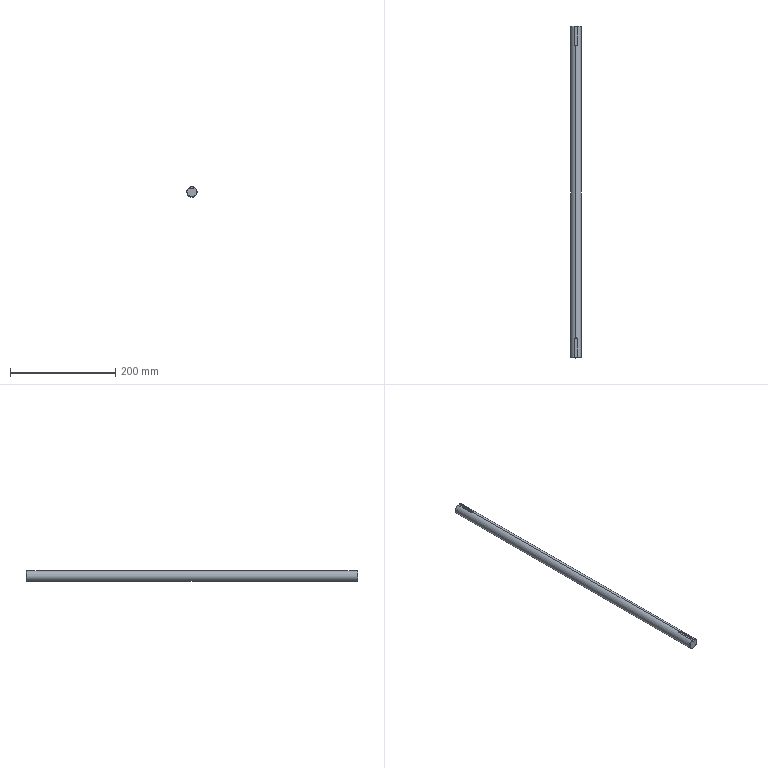Component | SolidWorks | ZL-11-09DriveShaft2-1 | 1 solid | 15 faces | box 20 x 630 x 20 mm | volume 196364 mm3 | plane 8 | cylinder 4 | cone 3 | commonest cylinder face diameters 20 x2 6 x2
build123d program:
from build123d import *

# Parameters (mm, degrees)
SKETCH1_R          = 10
EXTRUDE1_DEPTH     = 315
CUT_EXTRUDE1_DEPTH = 3.5
CHAMFER1_SIZE      = 1


with BuildPart() as part:
    # Sketch1 → Extrude1 (new, symmetric)
    with BuildSketch(Plane(origin=(0, 0, 0), x_dir=(1, 0, 0), z_dir=(0, 1, 0))):
        with Locations(Location((0, 0, 0), (0, 0, 270))):
            Circle(SKETCH1_R)
    extrude(amount=EXTRUDE1_DEPTH, both=True)

    # Sketch2 → Cut-Extrude1 (cut)
    with BuildSketch(Plane.XY.offset(10)):
        with BuildLine():
            Line((-3, 315), (3, 315))
            Line((3, 315), (3, 280))
            ThreePointArc((3, 280), (0, 277), (-3, 280))
            Line((-3, 280), (-3, 315))
        make_face()
    cut_extrude1 = extrude(amount=-CUT_EXTRUDE1_DEPTH, mode=Mode.SUBTRACT)

    # Mirror1: Cut-Extrude1 across plane
    add(cut_extrude1.mirror(Plane.ZX), mode=Mode.SUBTRACT)

    # Chamfer1
    chamfer1_edges = [part.edges().sort_by_distance(p)[0] for p in [
        (0, -315, -10),
        (0, 315, -10),
    ]]
    chamfer(chamfer1_edges, length=CHAMFER1_SIZE)


solid = part.part

# Placed as in the assembly
solid = solid.moved(Location((125.552, 443.22, 0.7679), (0, -1.419, 180)))
STEP:
#1=COLOUR_RGB('',0.7922,0.8196,0.9333);
#2=FILL_AREA_STYLE_COLOUR('',#1);
#3=FILL_AREA_STYLE('',(#2));
#4=SURFACE_STYLE_FILL_AREA(#3);
#5=SURFACE_SIDE_STYLE('',(#4));
#6=SURFACE_STYLE_USAGE(.BOTH.,#5);
#7=PRESENTATION_STYLE_ASSIGNMENT((#6));
#8=CARTESIAN_POINT('',(4.952,29.851,-0.324));
#9=VERTEX_POINT('',#8);
#10=CARTESIAN_POINT('',(4.817,29.851,0.3613));
#11=VERTEX_POINT('',#10);
#12=CARTESIAN_POINT('',(4.943,29.851,0.03023));
#13=DIRECTION('',(0.,1.,0.));
#14=DIRECTION('',(-0.02476,0.,0.9997));
#15=AXIS2_PLACEMENT_3D('',#12,#13,#14);
#16=CIRCLE('',#15,0.3543);
#17=EDGE_CURVE('',#9,#11,#16,.T.);
#18=ORIENTED_EDGE('',*,*,#17,.F.);
#19=CARTESIAN_POINT('',(4.953,29.812,-0.3633));
#20=VERTEX_POINT('',#19);
#21=CARTESIAN_POINT('',(4.952,29.851,-0.324));
#22=DIRECTION('',(0.01751,-0.7071,-0.7069));
#23=VECTOR('',#22,39.37);
#24=LINE('',#21,#23);
#25=EDGE_CURVE('',#9,#20,#24,.T.);
#26=ORIENTED_EDGE('',*,*,#25,.T.);
#27=CARTESIAN_POINT('',(4.816,29.812,0.4028));
#28=VERTEX_POINT('',#27);
#29=CARTESIAN_POINT('',(4.943,29.812,0.03023));
#30=DIRECTION('',(0.,-1.,0.));
#31=DIRECTION('',(-0.02476,0.,0.9997));
#32=AXIS2_PLACEMENT_3D('',#29,#30,#31);
#33=CIRCLE('',#32,0.3937);
#34=EDGE_CURVE('',#28,#20,#33,.T.);
#35=ORIENTED_EDGE('',*,*,#34,.F.);
#36=CARTESIAN_POINT('',(4.817,29.851,0.3613));
#37=CARTESIAN_POINT('',(4.816,29.838,0.3751));
#38=CARTESIAN_POINT('',(4.816,29.825,0.389));
#39=CARTESIAN_POINT('',(4.816,29.812,0.4028));
#40=B_SPLINE_CURVE_WITH_KNOTS('',3,(#36,#37,#38,#39),.UNSPECIFIED.,.F.,.F.,(4,4),(0.,0.001453),.UNSPECIFIED.);
#41=EDGE_CURVE('',#11,#28,#40,.T.);
#42=ORIENTED_EDGE('',*,*,#41,.F.);
#43=EDGE_LOOP('',(#18,#26,#35,#42));
#44=FACE_OUTER_BOUND('',#43,.T.);
#45=CARTESIAN_POINT('',(4.943,29.851,0.03023));
#46=DIRECTION('',(0.,-1.,0.));
#47=DIRECTION('',(0.02476,0.,-0.9997));
#48=AXIS2_PLACEMENT_3D('',#45,#46,#47);
#49=CONICAL_SURFACE('',#48,0.3543,0.7854);
#50=ADVANCED_FACE('',(#44),#49,.T.);
#51=CARTESIAN_POINT('',(5.052,28.473,0.4086));
#52=VERTEX_POINT('',#51);
#53=CARTESIAN_POINT('',(4.933,28.355,0.4238));
#54=VERTEX_POINT('',#53);
#55=CARTESIAN_POINT('',(5.052,28.473,0.4086));
#56=CARTESIAN_POINT('',(5.052,28.465,0.4086));
#57=CARTESIAN_POINT('',(5.051,28.458,0.4088));
#58=CARTESIAN_POINT('',(5.048,28.442,0.4097));
#59=CARTESIAN_POINT('',(5.046,28.435,0.4103));
#60=CARTESIAN_POINT('',(5.04,28.421,0.4119));
#61=CARTESIAN_POINT('',(5.036,28.414,0.4128));
#62=CARTESIAN_POINT('',(5.027,28.401,0.4148));
#63=CARTESIAN_POINT('',(5.022,28.395,0.4159));
#64=CARTESIAN_POINT('',(5.006,28.379,0.419));
#65=CARTESIAN_POINT('',(4.993,28.37,0.421));
#66=CARTESIAN_POINT('',(4.972,28.361,0.423));
#67=CARTESIAN_POINT('',(4.964,28.359,0.4234));
#68=CARTESIAN_POINT('',(4.949,28.356,0.424));
#69=CARTESIAN_POINT('',(4.941,28.355,0.424));
#70=CARTESIAN_POINT('',(4.933,28.355,0.4238));
#71=B_SPLINE_CURVE_WITH_KNOTS('',3,(#55,#56,#57,#58,#59,#60,#61,#62,#63,#64,#65,#66,#67,#68,#69,#70),.UNSPECIFIED.,.F.,.F.,(4,2,2,2,2,2,2,4),(0.,0.0005898,0.00118,0.001769,0.002359,0.003539,0.004128,0.004718),.UNSPECIFIED.);
#72=EDGE_CURVE('',#52,#54,#71,.T.);
#73=ORIENTED_EDGE('',*,*,#72,.T.);
#74=CARTESIAN_POINT('',(4.933,6.544,0.4238));
#75=VERTEX_POINT('',#74);
#76=CARTESIAN_POINT('',(4.933,29.851,0.4238));
#77=DIRECTION('',(0.,-1.,0.));
#78=VECTOR('',#77,39.37);
#79=LINE('',#76,#78);
#80=EDGE_CURVE('',#54,#75,#79,.T.);
#81=ORIENTED_EDGE('',*,*,#80,.T.);
#82=CARTESIAN_POINT('',(5.052,6.426,0.4086));
#83=VERTEX_POINT('',#82);
#84=CARTESIAN_POINT('',(5.052,6.426,0.4086));
#85=CARTESIAN_POINT('',(5.052,6.434,0.4086));
#86=CARTESIAN_POINT('',(5.051,6.442,0.4088));
#87=CARTESIAN_POINT('',(5.048,6.457,0.4097));
#88=CARTESIAN_POINT('',(5.046,6.464,0.4103));
#89=CARTESIAN_POINT('',(5.04,6.479,0.4119));
#90=CARTESIAN_POINT('',(5.036,6.485,0.4128));
#91=CARTESIAN_POINT('',(5.027,6.498,0.4148));
#92=CARTESIAN_POINT('',(5.022,6.504,0.4159));
#93=CARTESIAN_POINT('',(5.006,6.52,0.419));
#94=CARTESIAN_POINT('',(4.993,6.529,0.421));
#95=CARTESIAN_POINT('',(4.972,6.538,0.423));
#96=CARTESIAN_POINT('',(4.964,6.54,0.4234));
#97=CARTESIAN_POINT('',(4.949,6.543,0.424));
#98=CARTESIAN_POINT('',(4.941,6.544,0.424));
#99=CARTESIAN_POINT('',(4.933,6.544,0.4238));
#100=B_SPLINE_CURVE_WITH_KNOTS('',3,(#84,#85,#86,#87,#88,#89,#90,#91,#92,#93,#94,#95,#96,#97,#98,#99),.UNSPECIFIED.,.F.,.F.,(4,2,2,2,2,2,2,4),(0.,0.0005898,0.00118,0.001769,0.002359,0.003539,0.004128,0.004718),.UNSPECIFIED.);
#101=EDGE_CURVE('',#83,#75,#100,.T.);
#102=ORIENTED_EDGE('',*,*,#101,.F.);
#103=CARTESIAN_POINT('',(5.052,5.087,0.4086));
#104=VERTEX_POINT('',#103);
#105=CARTESIAN_POINT('',(5.052,29.851,0.4086));
#106=DIRECTION('',(0.,1.,0.));
#107=VECTOR('',#106,39.37);
#108=LINE('',#105,#107);
#109=EDGE_CURVE('',#104,#83,#108,.T.);
#110=ORIENTED_EDGE('',*,*,#109,.F.);
#111=CARTESIAN_POINT('',(4.953,5.087,-0.3633));
#112=VERTEX_POINT('',#111);
#113=CARTESIAN_POINT('',(4.943,5.087,0.03023));
#114=DIRECTION('',(0.,1.,0.));
#115=DIRECTION('',(-0.02476,0.,0.9997));
#116=AXIS2_PLACEMENT_3D('',#113,#114,#115);
#117=CIRCLE('',#116,0.3937);
#118=EDGE_CURVE('',#104,#112,#117,.T.);
#119=ORIENTED_EDGE('',*,*,#118,.T.);
#120=CARTESIAN_POINT('',(4.953,29.851,-0.3633));
#121=DIRECTION('',(0.,-1.,0.));
#122=VECTOR('',#121,39.37);
#123=LINE('',#120,#122);
#124=EDGE_CURVE('',#20,#112,#123,.T.);
#125=ORIENTED_EDGE('',*,*,#124,.F.);
#126=CARTESIAN_POINT('',(5.052,29.812,0.4086));
#127=VERTEX_POINT('',#126);
#128=CARTESIAN_POINT('',(4.943,29.812,0.03023));
#129=DIRECTION('',(0.,-1.,0.));
#130=DIRECTION('',(-0.02476,0.,0.9997));
#131=AXIS2_PLACEMENT_3D('',#128,#129,#130);
#132=CIRCLE('',#131,0.3937);
#133=EDGE_CURVE('',#20,#127,#132,.T.);
#134=ORIENTED_EDGE('',*,*,#133,.T.);
#135=CARTESIAN_POINT('',(5.052,29.851,0.4086));
#136=DIRECTION('',(0.,-1.,0.));
#137=VECTOR('',#136,39.37);
#138=LINE('',#135,#137);
#139=EDGE_CURVE('',#127,#52,#138,.T.);
#140=ORIENTED_EDGE('',*,*,#139,.T.);
#141=EDGE_LOOP('',(#73,#81,#102,#110,#119,#125,#134,#140));
#142=FACE_OUTER_BOUND('',#141,.T.);
#143=CARTESIAN_POINT('',(4.943,29.851,0.03023));
#144=DIRECTION('',(0.,-1.,0.));
#145=DIRECTION('',(0.02476,0.,-0.9997));
#146=AXIS2_PLACEMENT_3D('',#143,#144,#145);
#147=CYLINDRICAL_SURFACE('',#146,0.3937);
#148=ADVANCED_FACE('',(#142),#147,.T.);
#149=ORIENTED_EDGE('',*,*,#80,.F.);
#150=CARTESIAN_POINT('',(4.816,28.473,0.4028));
#151=VERTEX_POINT('',#150);
#152=CARTESIAN_POINT('',(4.933,28.355,0.4238));
#153=CARTESIAN_POINT('',(4.925,28.355,0.4236));
#154=CARTESIAN_POINT('',(4.918,28.356,0.4232));
#155=CARTESIAN_POINT('',(4.902,28.359,0.4219));
#156=CARTESIAN_POINT('',(4.895,28.361,0.4211));
#157=CARTESIAN_POINT('',(4.881,28.367,0.4191));
#158=CARTESIAN_POINT('',(4.874,28.371,0.4179));
#159=CARTESIAN_POINT('',(4.861,28.379,0.4154));
#160=CARTESIAN_POINT('',(4.855,28.384,0.4141));
#161=CARTESIAN_POINT('',(4.845,28.395,0.4115));
#162=CARTESIAN_POINT('',(4.84,28.401,0.4102));
#163=CARTESIAN_POINT('',(4.831,28.414,0.4078));
#164=CARTESIAN_POINT('',(4.828,28.421,0.4066));
#165=CARTESIAN_POINT('',(4.822,28.435,0.4048));
#166=CARTESIAN_POINT('',(4.819,28.442,0.404));
#167=CARTESIAN_POINT('',(4.816,28.458,0.403));
#168=CARTESIAN_POINT('',(4.816,28.465,0.4028));
#169=CARTESIAN_POINT('',(4.816,28.473,0.4028));
#170=B_SPLINE_CURVE_WITH_KNOTS('',3,(#152,#153,#154,#155,#156,#157,#158,#159,#160,#161,#162,#163,#164,#165,#166,#167,#168,#169),.UNSPECIFIED.,.F.,.F.,(4,2,2,2,2,2,2,2,4),(0.004718,0.005307,0.005896,0.006485,0.007074,0.007663,0.008252,0.008842,0.009431),.UNSPECIFIED.);
#171=EDGE_CURVE('',#54,#151,#170,.T.);
#172=ORIENTED_EDGE('',*,*,#171,.T.);
#173=CARTESIAN_POINT('',(4.816,29.851,0.4028));
#174=DIRECTION('',(0.,1.,0.));
#175=VECTOR('',#174,39.37);
#176=LINE('',#173,#175);
#177=EDGE_CURVE('',#151,#28,#176,.T.);
#178=ORIENTED_EDGE('',*,*,#177,.T.);
#179=ORIENTED_EDGE('',*,*,#34,.T.);
#180=ORIENTED_EDGE('',*,*,#124,.T.);
#181=CARTESIAN_POINT('',(4.816,5.087,0.4028));
#182=VERTEX_POINT('',#181);
#183=CARTESIAN_POINT('',(4.943,5.087,0.03023));
#184=DIRECTION('',(0.,1.,0.));
#185=DIRECTION('',(-0.02476,0.,0.9997));
#186=AXIS2_PLACEMENT_3D('',#183,#184,#185);
#187=CIRCLE('',#186,0.3937);
#188=EDGE_CURVE('',#112,#182,#187,.T.);
#189=ORIENTED_EDGE('',*,*,#188,.T.);
#190=CARTESIAN_POINT('',(4.816,6.426,0.4028));
#191=VERTEX_POINT('',#190);
#192=CARTESIAN_POINT('',(4.816,29.851,0.4028));
#193=DIRECTION('',(0.,-1.,0.));
#194=VECTOR('',#193,39.37);
#195=LINE('',#192,#194);
#196=EDGE_CURVE('',#191,#182,#195,.T.);
#197=ORIENTED_EDGE('',*,*,#196,.F.);
#198=CARTESIAN_POINT('',(4.933,6.544,0.4238));
#199=CARTESIAN_POINT('',(4.925,6.544,0.4236));
#200=CARTESIAN_POINT('',(4.918,6.543,0.4232));
#201=CARTESIAN_POINT('',(4.902,6.54,0.4219));
#202=CARTESIAN_POINT('',(4.895,6.538,0.4211));
#203=CARTESIAN_POINT('',(4.881,6.532,0.4191));
#204=CARTESIAN_POINT('',(4.874,6.528,0.4179));
#205=CARTESIAN_POINT('',(4.861,6.52,0.4154));
#206=CARTESIAN_POINT('',(4.855,6.515,0.4141));
#207=CARTESIAN_POINT('',(4.845,6.504,0.4115));
#208=CARTESIAN_POINT('',(4.84,6.498,0.4102));
#209=CARTESIAN_POINT('',(4.831,6.485,0.4078));
#210=CARTESIAN_POINT('',(4.828,6.478,0.4066));
#211=CARTESIAN_POINT('',(4.822,6.464,0.4048));
#212=CARTESIAN_POINT('',(4.819,6.457,0.404));
#213=CARTESIAN_POINT('',(4.816,6.442,0.403));
#214=CARTESIAN_POINT('',(4.816,6.434,0.4028));
#215=CARTESIAN_POINT('',(4.816,6.426,0.4028));
#216=B_SPLINE_CURVE_WITH_KNOTS('',3,(#198,#199,#200,#201,#202,#203,#204,#205,#206,#207,#208,#209,#210,#211,#212,#213,#214,#215),.UNSPECIFIED.,.F.,.F.,(4,2,2,2,2,2,2,2,4),(0.004718,0.005307,0.005896,0.006485,0.007074,0.007663,0.008252,0.008842,0.009431),.UNSPECIFIED.);
#217=EDGE_CURVE('',#75,#191,#216,.T.);
#218=ORIENTED_EDGE('',*,*,#217,.F.);
#219=EDGE_LOOP('',(#149,#172,#178,#179,#180,#189,#197,#218));
#220=FACE_OUTER_BOUND('',#219,.T.);
#221=CARTESIAN_POINT('',(4.943,29.851,0.03023));
#222=DIRECTION('',(0.,-1.,0.));
#223=DIRECTION('',(0.02476,0.,-0.9997));
#224=AXIS2_PLACEMENT_3D('',#221,#222,#223);
#225=CYLINDRICAL_SURFACE('',#224,0.3937);
#226=ADVANCED_FACE('',(#220),#225,.T.);
#227=CARTESIAN_POINT('',(4.819,5.048,0.2831));
#228=VERTEX_POINT('',#227);
#229=CARTESIAN_POINT('',(4.817,5.048,0.3613));
#230=VERTEX_POINT('',#229);
#231=CARTESIAN_POINT('',(4.819,5.048,0.2831));
#232=DIRECTION('',(-0.02476,0.,0.9997));
#233=VECTOR('',#232,39.37);
#234=LINE('',#231,#233);
#235=EDGE_CURVE('',#228,#230,#234,.T.);
#236=ORIENTED_EDGE('',*,*,#235,.T.);
#237=CARTESIAN_POINT('',(5.053,5.048,0.3671));
#238=VERTEX_POINT('',#237);
#239=CARTESIAN_POINT('',(4.943,5.048,0.03023));
#240=DIRECTION('',(0.,-1.,0.));
#241=DIRECTION('',(-0.02476,0.,0.9997));
#242=AXIS2_PLACEMENT_3D('',#239,#240,#241);
#243=CIRCLE('',#242,0.3543);
#244=EDGE_CURVE('',#230,#238,#243,.T.);
#245=ORIENTED_EDGE('',*,*,#244,.T.);
#246=CARTESIAN_POINT('',(5.055,5.048,0.289));
#247=VERTEX_POINT('',#246);
#248=CARTESIAN_POINT('',(5.055,5.048,0.289));
#249=DIRECTION('',(-0.02476,0.,0.9997));
#250=VECTOR('',#249,39.37);
#251=LINE('',#248,#250);
#252=EDGE_CURVE('',#247,#238,#251,.T.);
#253=ORIENTED_EDGE('',*,*,#252,.F.);
#254=CARTESIAN_POINT('',(4.819,5.048,0.2831));
#255=DIRECTION('',(-0.9997,0.,-0.02476));
#256=VECTOR('',#255,39.37);
#257=LINE('',#254,#256);
#258=EDGE_CURVE('',#247,#228,#257,.T.);
#259=ORIENTED_EDGE('',*,*,#258,.T.);
#260=EDGE_LOOP('',(#236,#245,#253,#259));
#261=FACE_OUTER_BOUND('',#260,.T.);
#262=CARTESIAN_POINT('',(4.943,5.048,0.03023));
#263=DIRECTION('',(0.,1.,0.));
#264=DIRECTION('',(-0.02476,0.,0.9997));
#265=AXIS2_PLACEMENT_3D('',#262,#263,#264);
#266=PLANE('',#265);
#267=ADVANCED_FACE('',(#261),#266,.F.);
#268=CARTESIAN_POINT('',(5.055,29.851,0.289));
#269=VERTEX_POINT('',#268);
#270=CARTESIAN_POINT('',(5.053,29.851,0.3671));
#271=VERTEX_POINT('',#270);
#272=CARTESIAN_POINT('',(5.055,29.851,0.289));
#273=DIRECTION('',(-0.02476,0.,0.9997));
#274=VECTOR('',#273,39.37);
#275=LINE('',#272,#274);
#276=EDGE_CURVE('',#269,#271,#275,.T.);
#277=ORIENTED_EDGE('',*,*,#276,.T.);
#278=CARTESIAN_POINT('',(4.943,29.851,0.03023));
#279=DIRECTION('',(0.,1.,0.));
#280=DIRECTION('',(-0.02476,0.,0.9997));
#281=AXIS2_PLACEMENT_3D('',#278,#279,#280);
#282=CIRCLE('',#281,0.3543);
#283=EDGE_CURVE('',#271,#9,#282,.T.);
#284=ORIENTED_EDGE('',*,*,#283,.T.);
#285=ORIENTED_EDGE('',*,*,#17,.T.);
#286=CARTESIAN_POINT('',(4.819,29.851,0.2831));
#287=VERTEX_POINT('',#286);
#288=CARTESIAN_POINT('',(4.819,29.851,0.2831));
#289=DIRECTION('',(-0.02476,0.,0.9997));
#290=VECTOR('',#289,39.37);
#291=LINE('',#288,#290);
#292=EDGE_CURVE('',#287,#11,#291,.T.);
#293=ORIENTED_EDGE('',*,*,#292,.F.);
#294=CARTESIAN_POINT('',(4.819,29.851,0.2831));
#295=DIRECTION('',(-0.9997,0.,-0.02476));
#296=VECTOR('',#295,39.37);
#297=LINE('',#294,#296);
#298=EDGE_CURVE('',#269,#287,#297,.T.);
#299=ORIENTED_EDGE('',*,*,#298,.F.);
#300=EDGE_LOOP('',(#277,#284,#285,#293,#299));
#301=FACE_OUTER_BOUND('',#300,.T.);
#302=CARTESIAN_POINT('',(4.943,29.851,0.03023));
#303=DIRECTION('',(0.,1.,0.));
#304=DIRECTION('',(-0.02476,0.,0.9997));
#305=AXIS2_PLACEMENT_3D('',#302,#303,#304);
#306=PLANE('',#305);
#307=ADVANCED_FACE('',(#301),#306,.T.);
#308=CARTESIAN_POINT('',(5.055,28.473,0.289));
#309=VERTEX_POINT('',#308);
#310=CARTESIAN_POINT('',(5.055,28.473,0.289));
#311=DIRECTION('',(-0.02476,0.,0.9997));
#312=VECTOR('',#311,39.37);
#313=LINE('',#310,#312);
#314=EDGE_CURVE('',#309,#52,#313,.T.);
#315=ORIENTED_EDGE('',*,*,#314,.F.);
#316=CARTESIAN_POINT('',(4.819,28.473,0.2831));
#317=VERTEX_POINT('',#316);
#318=CARTESIAN_POINT('',(4.937,28.473,0.2861));
#319=DIRECTION('',(-0.02476,0.,0.9997));
#320=DIRECTION('',(0.9997,0.,0.02476));
#321=AXIS2_PLACEMENT_3D('',#318,#319,#320);
#322=CIRCLE('',#321,0.1181);
#323=EDGE_CURVE('',#317,#309,#322,.T.);
#324=ORIENTED_EDGE('',*,*,#323,.F.);
#325=CARTESIAN_POINT('',(4.819,28.473,0.2831));
#326=DIRECTION('',(-0.02476,0.,0.9997));
#327=VECTOR('',#326,39.37);
#328=LINE('',#325,#327);
#329=EDGE_CURVE('',#317,#151,#328,.T.);
#330=ORIENTED_EDGE('',*,*,#329,.T.);
#331=ORIENTED_EDGE('',*,*,#171,.F.);
#332=ORIENTED_EDGE('',*,*,#72,.F.);
#333=EDGE_LOOP('',(#315,#324,#330,#331,#332));
#334=FACE_OUTER_BOUND('',#333,.T.);
#335=CARTESIAN_POINT('',(4.937,28.473,0.2861));
#336=DIRECTION('',(-0.02476,0.,0.9997));
#337=DIRECTION('',(0.9997,0.,0.02476));
#338=AXIS2_PLACEMENT_3D('',#335,#336,#337);
#339=CYLINDRICAL_SURFACE('',#338,0.1181);
#340=ADVANCED_FACE('',(#334),#339,.F.);
#341=ORIENTED_EDGE('',*,*,#292,.T.);
#342=ORIENTED_EDGE('',*,*,#41,.T.);
#343=ORIENTED_EDGE('',*,*,#177,.F.);
#344=ORIENTED_EDGE('',*,*,#329,.F.);
#345=CARTESIAN_POINT('',(4.819,29.851,0.2831));
#346=DIRECTION('',(0.,-1.,0.));
#347=VECTOR('',#346,39.37);
#348=LINE('',#345,#347);
#349=EDGE_CURVE('',#287,#317,#348,.T.);
#350=ORIENTED_EDGE('',*,*,#349,.F.);
#351=EDGE_LOOP('',(#341,#342,#343,#344,#350));
#352=FACE_OUTER_BOUND('',#351,.T.);
#353=CARTESIAN_POINT('',(4.819,29.851,0.2831));
#354=DIRECTION('',(-0.9997,-0.,-0.02476));
#355=DIRECTION('',(0.,-1.,0.));
#356=AXIS2_PLACEMENT_3D('',#353,#354,#355);
#357=PLANE('',#356);
#358=ADVANCED_FACE('',(#352),#357,.F.);
#359=ORIENTED_EDGE('',*,*,#139,.F.);
#360=CARTESIAN_POINT('',(5.052,29.812,0.4086));
#361=CARTESIAN_POINT('',(5.052,29.825,0.3948));
#362=CARTESIAN_POINT('',(5.052,29.838,0.381));
#363=CARTESIAN_POINT('',(5.053,29.851,0.3671));
#364=B_SPLINE_CURVE_WITH_KNOTS('',3,(#360,#361,#362,#363),.UNSPECIFIED.,.F.,.F.,(4,4),(0.,0.001453),.UNSPECIFIED.);
#365=EDGE_CURVE('',#127,#271,#364,.T.);
#366=ORIENTED_EDGE('',*,*,#365,.T.);
#367=ORIENTED_EDGE('',*,*,#276,.F.);
#368=CARTESIAN_POINT('',(5.055,29.851,0.289));
#369=DIRECTION('',(0.,1.,0.));
#370=VECTOR('',#369,39.37);
#371=LINE('',#368,#370);
#372=EDGE_CURVE('',#309,#269,#371,.T.);
#373=ORIENTED_EDGE('',*,*,#372,.F.);
#374=ORIENTED_EDGE('',*,*,#314,.T.);
#375=EDGE_LOOP('',(#359,#366,#367,#373,#374));
#376=FACE_OUTER_BOUND('',#375,.T.);
#377=CARTESIAN_POINT('',(5.055,29.851,0.289));
#378=DIRECTION('',(0.9997,-0.,0.02476));
#379=DIRECTION('',(0.,1.,0.));
#380=AXIS2_PLACEMENT_3D('',#377,#378,#379);
#381=PLANE('',#380);
#382=ADVANCED_FACE('',(#376),#381,.F.);
#383=ORIENTED_EDGE('',*,*,#349,.T.);
#384=ORIENTED_EDGE('',*,*,#323,.T.);
#385=ORIENTED_EDGE('',*,*,#372,.T.);
#386=ORIENTED_EDGE('',*,*,#298,.T.);
#387=EDGE_LOOP('',(#383,#384,#385,#386));
#388=FACE_OUTER_BOUND('',#387,.T.);
#389=CARTESIAN_POINT('',(4.937,28.473,0.2861));
#390=DIRECTION('',(-0.02476,0.,0.9997));
#391=DIRECTION('',(0.9997,0.,0.02476));
#392=AXIS2_PLACEMENT_3D('',#389,#390,#391);
#393=PLANE('',#392);
#394=ADVANCED_FACE('',(#388),#393,.T.);
#395=CARTESIAN_POINT('',(5.055,6.426,0.289));
#396=VERTEX_POINT('',#395);
#397=CARTESIAN_POINT('',(5.055,6.426,0.289));
#398=DIRECTION('',(-0.02476,0.,0.9997));
#399=VECTOR('',#398,39.37);
#400=LINE('',#397,#399);
#401=EDGE_CURVE('',#396,#83,#400,.T.);
#402=ORIENTED_EDGE('',*,*,#401,.T.);
#403=ORIENTED_EDGE('',*,*,#101,.T.);
#404=ORIENTED_EDGE('',*,*,#217,.T.);
#405=CARTESIAN_POINT('',(4.819,6.426,0.2831));
#406=VERTEX_POINT('',#405);
#407=CARTESIAN_POINT('',(4.819,6.426,0.2831));
#408=DIRECTION('',(-0.02476,0.,0.9997));
#409=VECTOR('',#408,39.37);
#410=LINE('',#407,#409);
#411=EDGE_CURVE('',#406,#191,#410,.T.);
#412=ORIENTED_EDGE('',*,*,#411,.F.);
#413=CARTESIAN_POINT('',(4.937,6.426,0.2861));
#414=DIRECTION('',(0.02476,0.,-0.9997));
#415=DIRECTION('',(0.9997,0.,0.02476));
#416=AXIS2_PLACEMENT_3D('',#413,#414,#415);
#417=CIRCLE('',#416,0.1181);
#418=EDGE_CURVE('',#406,#396,#417,.T.);
#419=ORIENTED_EDGE('',*,*,#418,.T.);
#420=EDGE_LOOP('',(#402,#403,#404,#412,#419));
#421=FACE_OUTER_BOUND('',#420,.T.);
#422=CARTESIAN_POINT('',(4.937,6.426,0.2861));
#423=DIRECTION('',(-0.02476,0.,0.9997));
#424=DIRECTION('',(0.9997,0.,0.02476));
#425=AXIS2_PLACEMENT_3D('',#422,#423,#424);
#426=CYLINDRICAL_SURFACE('',#425,0.1181);
#427=ADVANCED_FACE('',(#421),#426,.F.);
#428=ORIENTED_EDGE('',*,*,#196,.T.);
#429=CARTESIAN_POINT('',(4.816,5.087,0.4028));
#430=CARTESIAN_POINT('',(4.816,5.074,0.389));
#431=CARTESIAN_POINT('',(4.816,5.061,0.3751));
#432=CARTESIAN_POINT('',(4.817,5.048,0.3613));
#433=B_SPLINE_CURVE_WITH_KNOTS('',3,(#429,#430,#431,#432),.UNSPECIFIED.,.F.,.F.,(4,4),(0.,0.001453),.UNSPECIFIED.);
#434=EDGE_CURVE('',#182,#230,#433,.T.);
#435=ORIENTED_EDGE('',*,*,#434,.T.);
#436=ORIENTED_EDGE('',*,*,#235,.F.);
#437=CARTESIAN_POINT('',(4.819,5.048,0.2831));
#438=DIRECTION('',(0.,1.,0.));
#439=VECTOR('',#438,39.37);
#440=LINE('',#437,#439);
#441=EDGE_CURVE('',#228,#406,#440,.T.);
#442=ORIENTED_EDGE('',*,*,#441,.T.);
#443=ORIENTED_EDGE('',*,*,#411,.T.);
#444=EDGE_LOOP('',(#428,#435,#436,#442,#443));
#445=FACE_OUTER_BOUND('',#444,.T.);
#446=CARTESIAN_POINT('',(4.819,5.048,0.2831));
#447=DIRECTION('',(0.9997,-0.,0.02476));
#448=DIRECTION('',(0.,1.,0.));
#449=AXIS2_PLACEMENT_3D('',#446,#447,#448);
#450=PLANE('',#449);
#451=ADVANCED_FACE('',(#445),#450,.T.);
#452=ORIENTED_EDGE('',*,*,#252,.T.);
#453=CARTESIAN_POINT('',(5.053,5.048,0.3671));
#454=CARTESIAN_POINT('',(5.052,5.061,0.381));
#455=CARTESIAN_POINT('',(5.052,5.074,0.3948));
#456=CARTESIAN_POINT('',(5.052,5.087,0.4086));
#457=B_SPLINE_CURVE_WITH_KNOTS('',3,(#453,#454,#455,#456),.UNSPECIFIED.,.F.,.F.,(4,4),(0.,0.001453),.UNSPECIFIED.);
#458=EDGE_CURVE('',#238,#104,#457,.T.);
#459=ORIENTED_EDGE('',*,*,#458,.T.);
#460=ORIENTED_EDGE('',*,*,#109,.T.);
#461=ORIENTED_EDGE('',*,*,#401,.F.);
#462=CARTESIAN_POINT('',(5.055,5.048,0.289));
#463=DIRECTION('',(0.,-1.,0.));
#464=VECTOR('',#463,39.37);
#465=LINE('',#462,#464);
#466=EDGE_CURVE('',#396,#247,#465,.T.);
#467=ORIENTED_EDGE('',*,*,#466,.T.);
#468=EDGE_LOOP('',(#452,#459,#460,#461,#467));
#469=FACE_OUTER_BOUND('',#468,.T.);
#470=CARTESIAN_POINT('',(5.055,5.048,0.289));
#471=DIRECTION('',(-0.9997,-0.,-0.02476));
#472=DIRECTION('',(0.,-1.,0.));
#473=AXIS2_PLACEMENT_3D('',#470,#471,#472);
#474=PLANE('',#473);
#475=ADVANCED_FACE('',(#469),#474,.T.);
#476=ORIENTED_EDGE('',*,*,#441,.F.);
#477=ORIENTED_EDGE('',*,*,#258,.F.);
#478=ORIENTED_EDGE('',*,*,#466,.F.);
#479=ORIENTED_EDGE('',*,*,#418,.F.);
#480=EDGE_LOOP('',(#476,#477,#478,#479));
#481=FACE_OUTER_BOUND('',#480,.T.);
#482=CARTESIAN_POINT('',(4.937,6.426,0.2861));
#483=DIRECTION('',(-0.02476,0.,0.9997));
#484=DIRECTION('',(0.9997,0.,0.02476));
#485=AXIS2_PLACEMENT_3D('',#482,#483,#484);
#486=PLANE('',#485);
#487=ADVANCED_FACE('',(#481),#486,.T.);
#488=ORIENTED_EDGE('',*,*,#458,.F.);
#489=ORIENTED_EDGE('',*,*,#244,.F.);
#490=ORIENTED_EDGE('',*,*,#434,.F.);
#491=ORIENTED_EDGE('',*,*,#188,.F.);
#492=ORIENTED_EDGE('',*,*,#118,.F.);
#493=EDGE_LOOP('',(#488,#489,#490,#491,#492));
#494=FACE_OUTER_BOUND('',#493,.T.);
#495=CARTESIAN_POINT('',(4.943,5.087,0.03023));
#496=DIRECTION('',(0.,1.,0.));
#497=DIRECTION('',(-0.02476,0.,0.9997));
#498=AXIS2_PLACEMENT_3D('',#495,#496,#497);
#499=CONICAL_SURFACE('',#498,0.3937,0.7854);
#500=ADVANCED_FACE('',(#494),#499,.T.);
#501=ORIENTED_EDGE('',*,*,#25,.F.);
#502=ORIENTED_EDGE('',*,*,#283,.F.);
#503=ORIENTED_EDGE('',*,*,#365,.F.);
#504=ORIENTED_EDGE('',*,*,#133,.F.);
#505=EDGE_LOOP('',(#501,#502,#503,#504));
#506=FACE_OUTER_BOUND('',#505,.T.);
#507=CARTESIAN_POINT('',(4.943,29.851,0.03023));
#508=DIRECTION('',(0.,-1.,0.));
#509=DIRECTION('',(0.02476,0.,-0.9997));
#510=AXIS2_PLACEMENT_3D('',#507,#508,#509);
#511=CONICAL_SURFACE('',#510,0.3543,0.7854);
#512=ADVANCED_FACE('',(#506),#511,.T.);
#513=CLOSED_SHELL('',(#50,#148,#226,#267,#307,#340,#358,#382,#394,#427,#451,#475,#487,#500,#512));
#514=MANIFOLD_SOLID_BREP('',#513);
#515=STYLED_ITEM('',(#7),#514);
#516=(LENGTH_UNIT()NAMED_UNIT(*)SI_UNIT($,.METRE.));
#517=LENGTH_MEASURE_WITH_UNIT(LENGTH_MEASURE(0.0254),#516);
#518=DIMENSIONAL_EXPONENTS(1.,0.,0.,0.,0.,0.,0.);
#519=(CONVERSION_BASED_UNIT('',#517)LENGTH_UNIT()NAMED_UNIT(#518));
#520=UNCERTAINTY_MEASURE_WITH_UNIT(LENGTH_MEASURE(0.00001),#519,'','');
#521=(NAMED_UNIT(*)PLANE_ANGLE_UNIT()SI_UNIT($,.RADIAN.));
#522=(NAMED_UNIT(*)SI_UNIT($,.STERADIAN.)SOLID_ANGLE_UNIT());
#523=(GEOMETRIC_REPRESENTATION_CONTEXT(3)GLOBAL_UNCERTAINTY_ASSIGNED_CONTEXT((#520))GLOBAL_UNIT_ASSIGNED_CONTEXT((#519,#521,#522))REPRESENTATION_CONTEXT('',''));
#524=MECHANICAL_DESIGN_GEOMETRIC_PRESENTATION_REPRESENTATION('',(#515),#523);
#525=PRESENTATION_LAYER_ASSIGNMENT('','',(#515));
#526=CARTESIAN_POINT('',(0.,0.,0.));
#527=DIRECTION('',(0.,0.,1.));
#528=DIRECTION('',(1.,0.,0.));
#529=AXIS2_PLACEMENT_3D('',#526,#527,#528);
#530=(LENGTH_UNIT()NAMED_UNIT(*)SI_UNIT($,.METRE.));
#531=LENGTH_MEASURE_WITH_UNIT(LENGTH_MEASURE(0.0254),#530);
#532=DIMENSIONAL_EXPONENTS(1.,0.,0.,0.,0.,0.,0.);
#533=(CONVERSION_BASED_UNIT('',#531)LENGTH_UNIT()NAMED_UNIT(#532));
#534=UNCERTAINTY_MEASURE_WITH_UNIT(LENGTH_MEASURE(0.00001),#533,'','');
#535=(NAMED_UNIT(*)PLANE_ANGLE_UNIT()SI_UNIT($,.RADIAN.));
#536=(NAMED_UNIT(*)SI_UNIT($,.STERADIAN.)SOLID_ANGLE_UNIT());
#537=(GEOMETRIC_REPRESENTATION_CONTEXT(3)GLOBAL_UNCERTAINTY_ASSIGNED_CONTEXT((#534))GLOBAL_UNIT_ASSIGNED_CONTEXT((#533,#535,#536))REPRESENTATION_CONTEXT('',''));
#538=ADVANCED_BREP_SHAPE_REPRESENTATION('',(#514,#529),#537);